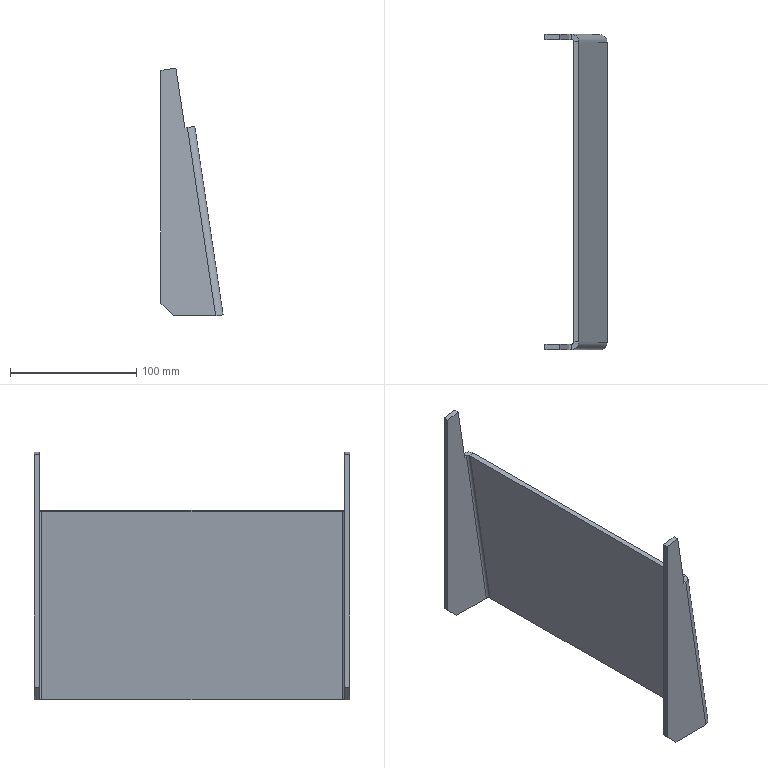Component | SolidWorks | THK-B1014SideStiffenerPlate-3 | 1 solid | 26 faces | box 49.3 x 250 x 196.5 mm | volume 195094 mm3 | plane 22 | cylinder 4 | commonest cylinder face diameters 12 x2 4 x2 | material Q235A
STEP:
#1=COLOUR_RGB('',0.7922,0.8196,0.9333);
#2=FILL_AREA_STYLE_COLOUR('',#1);
#3=FILL_AREA_STYLE('',(#2));
#4=SURFACE_STYLE_FILL_AREA(#3);
#5=SURFACE_SIDE_STYLE('',(#4));
#6=SURFACE_STYLE_USAGE(.BOTH.,#5);
#7=PRESENTATION_STYLE_ASSIGNMENT((#6));
#8=CARTESIAN_POINT('',(5.236,4.764,2.194));
#9=VERTEX_POINT('',#8);
#10=CARTESIAN_POINT('',(5.236,4.764,-5.079));
#11=VERTEX_POINT('',#10);
#12=CARTESIAN_POINT('',(5.236,4.764,-5.476));
#13=DIRECTION('',(0.,0.,-1.));
#14=VECTOR('',#13,39.37);
#15=LINE('',#12,#14);
#16=EDGE_CURVE('',#9,#11,#15,.T.);
#17=ORIENTED_EDGE('',*,*,#16,.T.);
#18=CARTESIAN_POINT('',(5.63,4.764,-5.472));
#19=VERTEX_POINT('',#18);
#20=CARTESIAN_POINT('',(5.63,4.764,-5.472));
#21=DIRECTION('',(0.7071,0.,-0.7071));
#22=VECTOR('',#21,39.37);
#23=LINE('',#20,#22);
#24=EDGE_CURVE('',#11,#19,#23,.T.);
#25=ORIENTED_EDGE('',*,*,#24,.T.);
#26=CARTESIAN_POINT('',(6.943,4.764,-5.472));
#27=VERTEX_POINT('',#26);
#28=CARTESIAN_POINT('',(7.183,4.764,-5.472));
#29=DIRECTION('',(1.,0.,0.));
#30=VECTOR('',#29,39.37);
#31=LINE('',#28,#30);
#32=EDGE_CURVE('',#19,#27,#31,.T.);
#33=ORIENTED_EDGE('',*,*,#32,.T.);
#34=CARTESIAN_POINT('',(6.062,4.764,0.4067));
#35=VERTEX_POINT('',#34);
#36=CARTESIAN_POINT('',(6.949,4.764,-5.511));
#37=DIRECTION('',(-0.1483,-0.,0.9889));
#38=VECTOR('',#37,39.37);
#39=LINE('',#36,#38);
#40=EDGE_CURVE('',#27,#35,#39,.T.);
#41=ORIENTED_EDGE('',*,*,#40,.T.);
#42=CARTESIAN_POINT('',(5.984,4.764,0.395));
#43=VERTEX_POINT('',#42);
#44=CARTESIAN_POINT('',(6.295,4.764,0.4417));
#45=DIRECTION('',(-0.9889,-0.,-0.1483));
#46=VECTOR('',#45,39.37);
#47=LINE('',#44,#46);
#48=EDGE_CURVE('',#35,#43,#47,.T.);
#49=ORIENTED_EDGE('',*,*,#48,.T.);
#50=CARTESIAN_POINT('',(5.703,4.764,2.264));
#51=VERTEX_POINT('',#50);
#52=CARTESIAN_POINT('',(6.871,4.764,-5.523));
#53=DIRECTION('',(-0.1483,-0.,0.9889));
#54=VECTOR('',#53,39.37);
#55=LINE('',#52,#54);
#56=EDGE_CURVE('',#43,#51,#55,.T.);
#57=ORIENTED_EDGE('',*,*,#56,.T.);
#58=CARTESIAN_POINT('',(6.015,4.764,2.311));
#59=DIRECTION('',(-0.9889,-0.,-0.1483));
#60=VECTOR('',#59,39.37);
#61=LINE('',#58,#60);
#62=EDGE_CURVE('',#51,#9,#61,.T.);
#63=ORIENTED_EDGE('',*,*,#62,.T.);
#64=EDGE_LOOP('',(#17,#25,#33,#41,#49,#57,#63));
#65=FACE_OUTER_BOUND('',#64,.T.);
#66=CARTESIAN_POINT('',(7.183,4.764,-5.476));
#67=DIRECTION('',(-0.,1.,0.));
#68=DIRECTION('',(0.9889,0.,0.1483));
#69=AXIS2_PLACEMENT_3D('',#66,#67,#68);
#70=PLANE('',#69);
#71=ADVANCED_FACE('',(#65),#70,.F.);
#72=CARTESIAN_POINT('',(6.943,4.921,-5.472));
#73=VERTEX_POINT('',#72);
#74=CARTESIAN_POINT('',(5.63,4.921,-5.472));
#75=VERTEX_POINT('',#74);
#76=CARTESIAN_POINT('',(6.943,4.921,-5.472));
#77=DIRECTION('',(-1.,-0.,-0.));
#78=VECTOR('',#77,39.37);
#79=LINE('',#76,#78);
#80=EDGE_CURVE('',#73,#75,#79,.T.);
#81=ORIENTED_EDGE('',*,*,#80,.T.);
#82=CARTESIAN_POINT('',(5.236,4.921,-5.079));
#83=VERTEX_POINT('',#82);
#84=CARTESIAN_POINT('',(6.408,4.921,-6.251));
#85=DIRECTION('',(-0.7071,-0.,0.7071));
#86=VECTOR('',#85,39.37);
#87=LINE('',#84,#86);
#88=EDGE_CURVE('',#75,#83,#87,.T.);
#89=ORIENTED_EDGE('',*,*,#88,.T.);
#90=CARTESIAN_POINT('',(5.236,4.921,2.194));
#91=VERTEX_POINT('',#90);
#92=CARTESIAN_POINT('',(5.236,4.921,-5.476));
#93=DIRECTION('',(0.,0.,-1.));
#94=VECTOR('',#93,39.37);
#95=LINE('',#92,#94);
#96=EDGE_CURVE('',#91,#83,#95,.T.);
#97=ORIENTED_EDGE('',*,*,#96,.F.);
#98=CARTESIAN_POINT('',(5.703,4.921,2.264));
#99=VERTEX_POINT('',#98);
#100=CARTESIAN_POINT('',(6.015,4.921,2.311));
#101=DIRECTION('',(-0.9889,-0.,-0.1483));
#102=VECTOR('',#101,39.37);
#103=LINE('',#100,#102);
#104=EDGE_CURVE('',#99,#91,#103,.T.);
#105=ORIENTED_EDGE('',*,*,#104,.F.);
#106=CARTESIAN_POINT('',(5.984,4.921,0.395));
#107=VERTEX_POINT('',#106);
#108=CARTESIAN_POINT('',(6.871,4.921,-5.523));
#109=DIRECTION('',(-0.1483,-0.,0.9889));
#110=VECTOR('',#109,39.37);
#111=LINE('',#108,#110);
#112=EDGE_CURVE('',#107,#99,#111,.T.);
#113=ORIENTED_EDGE('',*,*,#112,.F.);
#114=CARTESIAN_POINT('',(6.062,4.921,0.4067));
#115=VERTEX_POINT('',#114);
#116=CARTESIAN_POINT('',(6.295,4.921,0.4417));
#117=DIRECTION('',(-0.9889,-0.,-0.1483));
#118=VECTOR('',#117,39.37);
#119=LINE('',#116,#118);
#120=EDGE_CURVE('',#115,#107,#119,.T.);
#121=ORIENTED_EDGE('',*,*,#120,.F.);
#122=CARTESIAN_POINT('',(6.949,4.921,-5.511));
#123=DIRECTION('',(-0.1483,-0.,0.9889));
#124=VECTOR('',#123,39.37);
#125=LINE('',#122,#124);
#126=EDGE_CURVE('',#73,#115,#125,.T.);
#127=ORIENTED_EDGE('',*,*,#126,.F.);
#128=EDGE_LOOP('',(#81,#89,#97,#105,#113,#121,#127));
#129=FACE_OUTER_BOUND('',#128,.T.);
#130=CARTESIAN_POINT('',(7.183,4.921,-5.476));
#131=DIRECTION('',(-0.,1.,0.));
#132=DIRECTION('',(0.9889,0.,0.1483));
#133=AXIS2_PLACEMENT_3D('',#130,#131,#132);
#134=PLANE('',#133);
#135=ADVANCED_FACE('',(#129),#134,.T.);
#136=CARTESIAN_POINT('',(5.703,4.764,2.264));
#137=DIRECTION('',(-0.,1.,0.));
#138=VECTOR('',#137,39.37);
#139=LINE('',#136,#138);
#140=EDGE_CURVE('',#51,#99,#139,.T.);
#141=ORIENTED_EDGE('',*,*,#140,.T.);
#142=ORIENTED_EDGE('',*,*,#104,.T.);
#143=CARTESIAN_POINT('',(5.236,4.764,2.194));
#144=DIRECTION('',(-0.,1.,0.));
#145=VECTOR('',#144,39.37);
#146=LINE('',#143,#145);
#147=EDGE_CURVE('',#9,#91,#146,.T.);
#148=ORIENTED_EDGE('',*,*,#147,.F.);
#149=ORIENTED_EDGE('',*,*,#62,.F.);
#150=EDGE_LOOP('',(#141,#142,#148,#149));
#151=FACE_OUTER_BOUND('',#150,.T.);
#152=CARTESIAN_POINT('',(5.781,4.685,2.276));
#153=DIRECTION('',(0.1483,0.,-0.9889));
#154=DIRECTION('',(0.9889,0.,0.1483));
#155=AXIS2_PLACEMENT_3D('',#152,#153,#154);
#156=PLANE('',#155);
#157=ADVANCED_FACE('',(#151),#156,.F.);
#158=CARTESIAN_POINT('',(5.236,-4.921,2.194));
#159=VERTEX_POINT('',#158);
#160=CARTESIAN_POINT('',(5.703,-4.921,2.264));
#161=VERTEX_POINT('',#160);
#162=CARTESIAN_POINT('',(4.068,-4.921,2.019));
#163=DIRECTION('',(0.9889,0.,0.1483));
#164=VECTOR('',#163,39.37);
#165=LINE('',#162,#164);
#166=EDGE_CURVE('',#159,#161,#165,.T.);
#167=ORIENTED_EDGE('',*,*,#166,.T.);
#168=CARTESIAN_POINT('',(5.703,-4.764,2.264));
#169=VERTEX_POINT('',#168);
#170=CARTESIAN_POINT('',(5.703,-4.921,2.264));
#171=DIRECTION('',(-0.,1.,-0.));
#172=VECTOR('',#171,39.37);
#173=LINE('',#170,#172);
#174=EDGE_CURVE('',#161,#169,#173,.T.);
#175=ORIENTED_EDGE('',*,*,#174,.T.);
#176=CARTESIAN_POINT('',(5.236,-4.764,2.194));
#177=VERTEX_POINT('',#176);
#178=CARTESIAN_POINT('',(4.068,-4.764,2.019));
#179=DIRECTION('',(0.9889,0.,0.1483));
#180=VECTOR('',#179,39.37);
#181=LINE('',#178,#180);
#182=EDGE_CURVE('',#177,#169,#181,.T.);
#183=ORIENTED_EDGE('',*,*,#182,.F.);
#184=CARTESIAN_POINT('',(5.236,-4.764,2.194));
#185=DIRECTION('',(0.,-1.,0.));
#186=VECTOR('',#185,39.37);
#187=LINE('',#184,#186);
#188=EDGE_CURVE('',#177,#159,#187,.T.);
#189=ORIENTED_EDGE('',*,*,#188,.T.);
#190=EDGE_LOOP('',(#167,#175,#183,#189));
#191=FACE_OUTER_BOUND('',#190,.T.);
#192=CARTESIAN_POINT('',(5.859,-4.685,2.287));
#193=DIRECTION('',(-0.1483,-0.,0.9889));
#194=DIRECTION('',(-0.9889,-0.,-0.1483));
#195=AXIS2_PLACEMENT_3D('',#192,#193,#194);
#196=PLANE('',#195);
#197=ADVANCED_FACE('',(#191),#196,.T.);
#198=CARTESIAN_POINT('',(5.236,-4.921,-5.079));
#199=VERTEX_POINT('',#198);
#200=CARTESIAN_POINT('',(5.236,-4.921,-5.768));
#201=DIRECTION('',(-0.,0.,1.));
#202=VECTOR('',#201,39.37);
#203=LINE('',#200,#202);
#204=EDGE_CURVE('',#199,#159,#203,.T.);
#205=ORIENTED_EDGE('',*,*,#204,.F.);
#206=CARTESIAN_POINT('',(5.63,-4.921,-5.472));
#207=VERTEX_POINT('',#206);
#208=CARTESIAN_POINT('',(5.581,-4.921,-5.424));
#209=DIRECTION('',(0.7071,0.,-0.7071));
#210=VECTOR('',#209,39.37);
#211=LINE('',#208,#210);
#212=EDGE_CURVE('',#199,#207,#211,.T.);
#213=ORIENTED_EDGE('',*,*,#212,.T.);
#214=CARTESIAN_POINT('',(6.943,-4.921,-5.472));
#215=VERTEX_POINT('',#214);
#216=CARTESIAN_POINT('',(6.943,-4.921,-5.472));
#217=DIRECTION('',(-1.,-0.,-0.));
#218=VECTOR('',#217,39.37);
#219=LINE('',#216,#218);
#220=EDGE_CURVE('',#215,#207,#219,.T.);
#221=ORIENTED_EDGE('',*,*,#220,.F.);
#222=CARTESIAN_POINT('',(6.062,-4.921,0.4067));
#223=VERTEX_POINT('',#222);
#224=CARTESIAN_POINT('',(6.949,-4.921,-5.511));
#225=DIRECTION('',(-0.1483,-0.,0.9889));
#226=VECTOR('',#225,39.37);
#227=LINE('',#224,#226);
#228=EDGE_CURVE('',#215,#223,#227,.T.);
#229=ORIENTED_EDGE('',*,*,#228,.T.);
#230=CARTESIAN_POINT('',(5.984,-4.921,0.395));
#231=VERTEX_POINT('',#230);
#232=CARTESIAN_POINT('',(5.984,-4.921,0.395));
#233=DIRECTION('',(0.9889,0.,0.1483));
#234=VECTOR('',#233,39.37);
#235=LINE('',#232,#234);
#236=EDGE_CURVE('',#231,#223,#235,.T.);
#237=ORIENTED_EDGE('',*,*,#236,.F.);
#238=CARTESIAN_POINT('',(5.703,-4.921,2.264));
#239=DIRECTION('',(0.1483,0.,-0.9889));
#240=VECTOR('',#239,39.37);
#241=LINE('',#238,#240);
#242=EDGE_CURVE('',#161,#231,#241,.T.);
#243=ORIENTED_EDGE('',*,*,#242,.F.);
#244=ORIENTED_EDGE('',*,*,#166,.F.);
#245=EDGE_LOOP('',(#205,#213,#221,#229,#237,#243,#244));
#246=FACE_OUTER_BOUND('',#245,.T.);
#247=CARTESIAN_POINT('',(5.236,-4.921,-5.768));
#248=DIRECTION('',(0.,-1.,0.));
#249=DIRECTION('',(0.1483,0.,-0.9889));
#250=AXIS2_PLACEMENT_3D('',#247,#248,#249);
#251=PLANE('',#250);
#252=ADVANCED_FACE('',(#246),#251,.T.);
#253=CARTESIAN_POINT('',(6.943,-4.764,-5.472));
#254=VERTEX_POINT('',#253);
#255=CARTESIAN_POINT('',(5.63,-4.764,-5.472));
#256=VERTEX_POINT('',#255);
#257=CARTESIAN_POINT('',(5.236,-4.764,-5.472));
#258=DIRECTION('',(-1.,-0.,-0.));
#259=VECTOR('',#258,39.37);
#260=LINE('',#257,#259);
#261=EDGE_CURVE('',#254,#256,#260,.T.);
#262=ORIENTED_EDGE('',*,*,#261,.T.);
#263=CARTESIAN_POINT('',(5.236,-4.764,-5.079));
#264=VERTEX_POINT('',#263);
#265=CARTESIAN_POINT('',(5.63,-4.764,-5.472));
#266=DIRECTION('',(-0.7071,-0.,0.7071));
#267=VECTOR('',#266,39.37);
#268=LINE('',#265,#267);
#269=EDGE_CURVE('',#256,#264,#268,.T.);
#270=ORIENTED_EDGE('',*,*,#269,.T.);
#271=CARTESIAN_POINT('',(5.236,-4.764,-5.768));
#272=DIRECTION('',(-0.,0.,1.));
#273=VECTOR('',#272,39.37);
#274=LINE('',#271,#273);
#275=EDGE_CURVE('',#264,#177,#274,.T.);
#276=ORIENTED_EDGE('',*,*,#275,.T.);
#277=ORIENTED_EDGE('',*,*,#182,.T.);
#278=CARTESIAN_POINT('',(5.984,-4.764,0.395));
#279=VERTEX_POINT('',#278);
#280=CARTESIAN_POINT('',(6.871,-4.764,-5.523));
#281=DIRECTION('',(0.1483,0.,-0.9889));
#282=VECTOR('',#281,39.37);
#283=LINE('',#280,#282);
#284=EDGE_CURVE('',#169,#279,#283,.T.);
#285=ORIENTED_EDGE('',*,*,#284,.T.);
#286=CARTESIAN_POINT('',(6.062,-4.764,0.4067));
#287=VERTEX_POINT('',#286);
#288=CARTESIAN_POINT('',(4.349,-4.764,0.1497));
#289=DIRECTION('',(0.9889,0.,0.1483));
#290=VECTOR('',#289,39.37);
#291=LINE('',#288,#290);
#292=EDGE_CURVE('',#279,#287,#291,.T.);
#293=ORIENTED_EDGE('',*,*,#292,.T.);
#294=CARTESIAN_POINT('',(6.949,-4.764,-5.511));
#295=DIRECTION('',(-0.1483,-0.,0.9889));
#296=VECTOR('',#295,39.37);
#297=LINE('',#294,#296);
#298=EDGE_CURVE('',#254,#287,#297,.T.);
#299=ORIENTED_EDGE('',*,*,#298,.F.);
#300=EDGE_LOOP('',(#262,#270,#276,#277,#285,#293,#299));
#301=FACE_OUTER_BOUND('',#300,.T.);
#302=CARTESIAN_POINT('',(5.236,-4.764,-5.768));
#303=DIRECTION('',(0.,-1.,0.));
#304=DIRECTION('',(0.1483,0.,-0.9889));
#305=AXIS2_PLACEMENT_3D('',#302,#303,#304);
#306=PLANE('',#305);
#307=ADVANCED_FACE('',(#301),#306,.F.);
#308=CARTESIAN_POINT('',(7.177,4.685,-5.437));
#309=VERTEX_POINT('',#308);
#310=CARTESIAN_POINT('',(6.943,4.685,-5.472));
#311=DIRECTION('',(0.1483,0.,-0.9889));
#312=DIRECTION('',(-0.9889,-0.,-0.1483));
#313=AXIS2_PLACEMENT_3D('',#310,#311,#312);
#314=CIRCLE('',#313,0.2362);
#315=EDGE_CURVE('',#73,#309,#314,.T.);
#316=ORIENTED_EDGE('',*,*,#315,.F.);
#317=ORIENTED_EDGE('',*,*,#126,.T.);
#318=CARTESIAN_POINT('',(6.295,4.685,0.4417));
#319=VERTEX_POINT('',#318);
#320=CARTESIAN_POINT('',(6.062,4.685,0.4067));
#321=DIRECTION('',(-0.1483,-0.,0.9889));
#322=DIRECTION('',(0.9889,0.,0.1483));
#323=AXIS2_PLACEMENT_3D('',#320,#321,#322);
#324=CIRCLE('',#323,0.2362);
#325=EDGE_CURVE('',#319,#115,#324,.T.);
#326=ORIENTED_EDGE('',*,*,#325,.F.);
#327=CARTESIAN_POINT('',(7.183,4.685,-5.476));
#328=DIRECTION('',(-0.1483,-0.,0.9889));
#329=VECTOR('',#328,39.37);
#330=LINE('',#327,#329);
#331=EDGE_CURVE('',#309,#319,#330,.T.);
#332=ORIENTED_EDGE('',*,*,#331,.F.);
#333=EDGE_LOOP('',(#316,#317,#326,#332));
#334=FACE_OUTER_BOUND('',#333,.T.);
#335=CARTESIAN_POINT('',(6.949,4.685,-5.511));
#336=DIRECTION('',(-0.1483,-0.,0.9889));
#337=DIRECTION('',(-0.9889,-0.,-0.1483));
#338=AXIS2_PLACEMENT_3D('',#335,#336,#337);
#339=CYLINDRICAL_SURFACE('',#338,0.2362);
#340=ADVANCED_FACE('',(#334),#339,.T.);
#341=CARTESIAN_POINT('',(7.177,-4.685,-5.437));
#342=VERTEX_POINT('',#341);
#343=CARTESIAN_POINT('',(7.177,4.921,-5.437));
#344=DIRECTION('',(0.,-1.,0.));
#345=VECTOR('',#344,39.37);
#346=LINE('',#343,#345);
#347=EDGE_CURVE('',#309,#342,#346,.T.);
#348=ORIENTED_EDGE('',*,*,#347,.F.);
#349=ORIENTED_EDGE('',*,*,#331,.T.);
#350=CARTESIAN_POINT('',(6.295,-4.685,0.4417));
#351=VERTEX_POINT('',#350);
#352=CARTESIAN_POINT('',(6.295,4.921,0.4417));
#353=DIRECTION('',(0.,-1.,0.));
#354=VECTOR('',#353,39.37);
#355=LINE('',#352,#354);
#356=EDGE_CURVE('',#319,#351,#355,.T.);
#357=ORIENTED_EDGE('',*,*,#356,.T.);
#358=CARTESIAN_POINT('',(7.183,-4.685,-5.476));
#359=DIRECTION('',(-0.1483,-0.,0.9889));
#360=VECTOR('',#359,39.37);
#361=LINE('',#358,#360);
#362=EDGE_CURVE('',#342,#351,#361,.T.);
#363=ORIENTED_EDGE('',*,*,#362,.F.);
#364=EDGE_LOOP('',(#348,#349,#357,#363));
#365=FACE_OUTER_BOUND('',#364,.T.);
#366=CARTESIAN_POINT('',(7.183,-4.921,-5.476));
#367=DIRECTION('',(0.9889,0.,0.1483));
#368=DIRECTION('',(0.,-1.,-0.));
#369=AXIS2_PLACEMENT_3D('',#366,#367,#368);
#370=PLANE('',#369);
#371=ADVANCED_FACE('',(#365),#370,.T.);
#372=CARTESIAN_POINT('',(6.943,-4.685,-5.472));
#373=DIRECTION('',(0.1483,0.,-0.9889));
#374=DIRECTION('',(-0.9889,-0.,-0.1483));
#375=AXIS2_PLACEMENT_3D('',#372,#373,#374);
#376=CIRCLE('',#375,0.2362);
#377=EDGE_CURVE('',#342,#215,#376,.T.);
#378=ORIENTED_EDGE('',*,*,#377,.F.);
#379=ORIENTED_EDGE('',*,*,#362,.T.);
#380=CARTESIAN_POINT('',(6.062,-4.685,0.4067));
#381=DIRECTION('',(-0.1483,-0.,0.9889));
#382=DIRECTION('',(0.9889,0.,0.1483));
#383=AXIS2_PLACEMENT_3D('',#380,#381,#382);
#384=CIRCLE('',#383,0.2362);
#385=EDGE_CURVE('',#223,#351,#384,.T.);
#386=ORIENTED_EDGE('',*,*,#385,.F.);
#387=ORIENTED_EDGE('',*,*,#228,.F.);
#388=EDGE_LOOP('',(#378,#379,#386,#387));
#389=FACE_OUTER_BOUND('',#388,.T.);
#390=CARTESIAN_POINT('',(6.949,-4.685,-5.511));
#391=DIRECTION('',(-0.1483,-0.,0.9889));
#392=DIRECTION('',(-0.9889,-0.,-0.1483));
#393=AXIS2_PLACEMENT_3D('',#390,#391,#392);
#394=CYLINDRICAL_SURFACE('',#393,0.2362);
#395=ADVANCED_FACE('',(#389),#394,.T.);
#396=CARTESIAN_POINT('',(7.021,-4.685,-5.461));
#397=VERTEX_POINT('',#396);
#398=CARTESIAN_POINT('',(6.14,-4.685,0.4183));
#399=VERTEX_POINT('',#398);
#400=CARTESIAN_POINT('',(7.027,-4.685,-5.5));
#401=DIRECTION('',(-0.1483,-0.,0.9889));
#402=VECTOR('',#401,39.37);
#403=LINE('',#400,#402);
#404=EDGE_CURVE('',#397,#399,#403,.T.);
#405=ORIENTED_EDGE('',*,*,#404,.F.);
#406=CARTESIAN_POINT('',(6.943,-4.685,-5.472));
#407=DIRECTION('',(0.1483,0.,-0.9889));
#408=DIRECTION('',(-0.9889,0.,-0.1483));
#409=AXIS2_PLACEMENT_3D('',#406,#407,#408);
#410=CIRCLE('',#409,0.07874);
#411=EDGE_CURVE('',#397,#254,#410,.T.);
#412=ORIENTED_EDGE('',*,*,#411,.T.);
#413=ORIENTED_EDGE('',*,*,#298,.T.);
#414=CARTESIAN_POINT('',(6.062,-4.685,0.4067));
#415=DIRECTION('',(-0.1483,-0.,0.9889));
#416=DIRECTION('',(-0.9889,0.,-0.1483));
#417=AXIS2_PLACEMENT_3D('',#414,#415,#416);
#418=CIRCLE('',#417,0.07874);
#419=EDGE_CURVE('',#287,#399,#418,.T.);
#420=ORIENTED_EDGE('',*,*,#419,.T.);
#421=EDGE_LOOP('',(#405,#412,#413,#420));
#422=FACE_OUTER_BOUND('',#421,.T.);
#423=CARTESIAN_POINT('',(6.949,-4.685,-5.511));
#424=DIRECTION('',(-0.1483,-0.,0.9889));
#425=DIRECTION('',(-0.9889,0.,-0.1483));
#426=AXIS2_PLACEMENT_3D('',#423,#424,#425);
#427=CYLINDRICAL_SURFACE('',#426,0.07874);
#428=ADVANCED_FACE('',(#422),#427,.F.);
#429=CARTESIAN_POINT('',(7.021,4.685,-5.461));
#430=VERTEX_POINT('',#429);
#431=CARTESIAN_POINT('',(6.14,4.685,0.4183));
#432=VERTEX_POINT('',#431);
#433=CARTESIAN_POINT('',(7.027,4.685,-5.5));
#434=DIRECTION('',(-0.1483,-0.,0.9889));
#435=VECTOR('',#434,39.37);
#436=LINE('',#433,#435);
#437=EDGE_CURVE('',#430,#432,#436,.T.);
#438=ORIENTED_EDGE('',*,*,#437,.F.);
#439=CARTESIAN_POINT('',(7.021,-4.921,-5.461));
#440=DIRECTION('',(0.,-1.,-0.));
#441=VECTOR('',#440,39.37);
#442=LINE('',#439,#441);
#443=EDGE_CURVE('',#430,#397,#442,.T.);
#444=ORIENTED_EDGE('',*,*,#443,.T.);
#445=ORIENTED_EDGE('',*,*,#404,.T.);
#446=CARTESIAN_POINT('',(6.14,-4.921,0.4183));
#447=DIRECTION('',(0.,-1.,-0.));
#448=VECTOR('',#447,39.37);
#449=LINE('',#446,#448);
#450=EDGE_CURVE('',#432,#399,#449,.T.);
#451=ORIENTED_EDGE('',*,*,#450,.F.);
#452=EDGE_LOOP('',(#438,#444,#445,#451));
#453=FACE_OUTER_BOUND('',#452,.T.);
#454=CARTESIAN_POINT('',(7.027,-4.921,-5.5));
#455=DIRECTION('',(0.9889,0.,0.1483));
#456=DIRECTION('',(0.,-1.,-0.));
#457=AXIS2_PLACEMENT_3D('',#454,#455,#456);
#458=PLANE('',#457);
#459=ADVANCED_FACE('',(#453),#458,.F.);
#460=ORIENTED_EDGE('',*,*,#40,.F.);
#461=CARTESIAN_POINT('',(6.943,4.685,-5.472));
#462=DIRECTION('',(0.1483,0.,-0.9889));
#463=DIRECTION('',(-0.9889,0.,-0.1483));
#464=AXIS2_PLACEMENT_3D('',#461,#462,#463);
#465=CIRCLE('',#464,0.07874);
#466=EDGE_CURVE('',#27,#430,#465,.T.);
#467=ORIENTED_EDGE('',*,*,#466,.T.);
#468=ORIENTED_EDGE('',*,*,#437,.T.);
#469=CARTESIAN_POINT('',(6.062,4.685,0.4067));
#470=DIRECTION('',(-0.1483,-0.,0.9889));
#471=DIRECTION('',(-0.9889,0.,-0.1483));
#472=AXIS2_PLACEMENT_3D('',#469,#470,#471);
#473=CIRCLE('',#472,0.07874);
#474=EDGE_CURVE('',#432,#35,#473,.T.);
#475=ORIENTED_EDGE('',*,*,#474,.T.);
#476=EDGE_LOOP('',(#460,#467,#468,#475));
#477=FACE_OUTER_BOUND('',#476,.T.);
#478=CARTESIAN_POINT('',(6.949,4.685,-5.511));
#479=DIRECTION('',(-0.1483,-0.,0.9889));
#480=DIRECTION('',(-0.9889,0.,-0.1483));
#481=AXIS2_PLACEMENT_3D('',#478,#479,#480);
#482=CYLINDRICAL_SURFACE('',#481,0.07874);
#483=ADVANCED_FACE('',(#477),#482,.F.);
#484=ORIENTED_EDGE('',*,*,#275,.F.);
#485=CARTESIAN_POINT('',(5.236,-4.921,-5.079));
#486=DIRECTION('',(0.,-1.,0.));
#487=VECTOR('',#486,39.37);
#488=LINE('',#485,#487);
#489=EDGE_CURVE('',#264,#199,#488,.T.);
#490=ORIENTED_EDGE('',*,*,#489,.T.);
#491=ORIENTED_EDGE('',*,*,#204,.T.);
#492=ORIENTED_EDGE('',*,*,#188,.F.);
#493=EDGE_LOOP('',(#484,#490,#491,#492));
#494=FACE_OUTER_BOUND('',#493,.T.);
#495=CARTESIAN_POINT('',(5.236,-4.764,-5.768));
#496=DIRECTION('',(1.,0.,0.));
#497=DIRECTION('',(-0.,0.,1.));
#498=AXIS2_PLACEMENT_3D('',#495,#496,#497);
#499=PLANE('',#498);
#500=ADVANCED_FACE('',(#494),#499,.F.);
#501=ORIENTED_EDGE('',*,*,#96,.T.);
#502=CARTESIAN_POINT('',(5.236,4.764,-5.079));
#503=DIRECTION('',(0.,-1.,0.));
#504=VECTOR('',#503,39.37);
#505=LINE('',#502,#504);
#506=EDGE_CURVE('',#83,#11,#505,.T.);
#507=ORIENTED_EDGE('',*,*,#506,.T.);
#508=ORIENTED_EDGE('',*,*,#16,.F.);
#509=ORIENTED_EDGE('',*,*,#147,.T.);
#510=EDGE_LOOP('',(#501,#507,#508,#509));
#511=FACE_OUTER_BOUND('',#510,.T.);
#512=CARTESIAN_POINT('',(5.236,4.764,-5.476));
#513=DIRECTION('',(1.,0.,0.));
#514=DIRECTION('',(0.,0.,-1.));
#515=AXIS2_PLACEMENT_3D('',#512,#513,#514);
#516=PLANE('',#515);
#517=ADVANCED_FACE('',(#511),#516,.F.);
#518=ORIENTED_EDGE('',*,*,#140,.F.);
#519=ORIENTED_EDGE('',*,*,#56,.F.);
#520=CARTESIAN_POINT('',(5.984,4.764,0.395));
#521=DIRECTION('',(-0.,1.,0.));
#522=VECTOR('',#521,39.37);
#523=LINE('',#520,#522);
#524=EDGE_CURVE('',#43,#107,#523,.T.);
#525=ORIENTED_EDGE('',*,*,#524,.T.);
#526=ORIENTED_EDGE('',*,*,#112,.T.);
#527=EDGE_LOOP('',(#518,#519,#525,#526));
#528=FACE_OUTER_BOUND('',#527,.T.);
#529=CARTESIAN_POINT('',(6.871,4.764,-5.523));
#530=DIRECTION('',(-0.9889,-0.,-0.1483));
#531=DIRECTION('',(-0.1483,-0.,0.9889));
#532=AXIS2_PLACEMENT_3D('',#529,#530,#531);
#533=PLANE('',#532);
#534=ADVANCED_FACE('',(#528),#533,.F.);
#535=ORIENTED_EDGE('',*,*,#524,.F.);
#536=ORIENTED_EDGE('',*,*,#48,.F.);
#537=CARTESIAN_POINT('',(6.062,4.764,0.4067));
#538=DIRECTION('',(-0.,1.,0.));
#539=VECTOR('',#538,39.37);
#540=LINE('',#537,#539);
#541=EDGE_CURVE('',#35,#115,#540,.T.);
#542=ORIENTED_EDGE('',*,*,#541,.T.);
#543=ORIENTED_EDGE('',*,*,#120,.T.);
#544=EDGE_LOOP('',(#535,#536,#542,#543));
#545=FACE_OUTER_BOUND('',#544,.T.);
#546=CARTESIAN_POINT('',(6.295,4.764,0.4417));
#547=DIRECTION('',(0.1483,0.,-0.9889));
#548=DIRECTION('',(-0.9889,-0.,-0.1483));
#549=AXIS2_PLACEMENT_3D('',#546,#547,#548);
#550=PLANE('',#549);
#551=ADVANCED_FACE('',(#545),#550,.F.);
#552=ORIENTED_EDGE('',*,*,#356,.F.);
#553=CARTESIAN_POINT('',(6.295,4.685,0.4417));
#554=DIRECTION('',(-0.9889,-0.,-0.1483));
#555=VECTOR('',#554,39.37);
#556=LINE('',#553,#555);
#557=EDGE_CURVE('',#319,#432,#556,.T.);
#558=ORIENTED_EDGE('',*,*,#557,.T.);
#559=ORIENTED_EDGE('',*,*,#450,.T.);
#560=CARTESIAN_POINT('',(6.295,-4.685,0.4417));
#561=DIRECTION('',(-0.9889,-0.,-0.1483));
#562=VECTOR('',#561,39.37);
#563=LINE('',#560,#562);
#564=EDGE_CURVE('',#351,#399,#563,.T.);
#565=ORIENTED_EDGE('',*,*,#564,.F.);
#566=EDGE_LOOP('',(#552,#558,#559,#565));
#567=FACE_OUTER_BOUND('',#566,.T.);
#568=CARTESIAN_POINT('',(6.295,4.921,0.4417));
#569=DIRECTION('',(-0.1483,-0.,0.9889));
#570=DIRECTION('',(0.,-1.,0.));
#571=AXIS2_PLACEMENT_3D('',#568,#569,#570);
#572=PLANE('',#571);
#573=ADVANCED_FACE('',(#567),#572,.T.);
#574=ORIENTED_EDGE('',*,*,#174,.F.);
#575=ORIENTED_EDGE('',*,*,#242,.T.);
#576=CARTESIAN_POINT('',(5.984,-4.921,0.395));
#577=DIRECTION('',(-0.,1.,-0.));
#578=VECTOR('',#577,39.37);
#579=LINE('',#576,#578);
#580=EDGE_CURVE('',#231,#279,#579,.T.);
#581=ORIENTED_EDGE('',*,*,#580,.T.);
#582=ORIENTED_EDGE('',*,*,#284,.F.);
#583=EDGE_LOOP('',(#574,#575,#581,#582));
#584=FACE_OUTER_BOUND('',#583,.T.);
#585=CARTESIAN_POINT('',(5.703,-4.921,2.264));
#586=DIRECTION('',(-0.9889,-0.,-0.1483));
#587=DIRECTION('',(0.1483,0.,-0.9889));
#588=AXIS2_PLACEMENT_3D('',#585,#586,#587);
#589=PLANE('',#588);
#590=ADVANCED_FACE('',(#584),#589,.F.);
#591=ORIENTED_EDGE('',*,*,#236,.T.);
#592=CARTESIAN_POINT('',(6.062,-4.921,0.4067));
#593=DIRECTION('',(-0.,1.,-0.));
#594=VECTOR('',#593,39.37);
#595=LINE('',#592,#594);
#596=EDGE_CURVE('',#223,#287,#595,.T.);
#597=ORIENTED_EDGE('',*,*,#596,.T.);
#598=ORIENTED_EDGE('',*,*,#292,.F.);
#599=ORIENTED_EDGE('',*,*,#580,.F.);
#600=EDGE_LOOP('',(#591,#597,#598,#599));
#601=FACE_OUTER_BOUND('',#600,.T.);
#602=CARTESIAN_POINT('',(5.984,-4.921,0.395));
#603=DIRECTION('',(0.1483,0.,-0.9889));
#604=DIRECTION('',(0.9889,0.,0.1483));
#605=AXIS2_PLACEMENT_3D('',#602,#603,#604);
#606=PLANE('',#605);
#607=ADVANCED_FACE('',(#601),#606,.F.);
#608=ORIENTED_EDGE('',*,*,#385,.T.);
#609=ORIENTED_EDGE('',*,*,#564,.T.);
#610=ORIENTED_EDGE('',*,*,#419,.F.);
#611=ORIENTED_EDGE('',*,*,#596,.F.);
#612=EDGE_LOOP('',(#608,#609,#610,#611));
#613=FACE_OUTER_BOUND('',#612,.T.);
#614=CARTESIAN_POINT('',(6.062,-4.685,0.4067));
#615=DIRECTION('',(-0.1483,-0.,0.9889));
#616=DIRECTION('',(-0.9889,-0.,-0.1483));
#617=AXIS2_PLACEMENT_3D('',#614,#615,#616);
#618=PLANE('',#617);
#619=ADVANCED_FACE('',(#613),#618,.T.);
#620=ORIENTED_EDGE('',*,*,#325,.T.);
#621=ORIENTED_EDGE('',*,*,#541,.F.);
#622=ORIENTED_EDGE('',*,*,#474,.F.);
#623=ORIENTED_EDGE('',*,*,#557,.F.);
#624=EDGE_LOOP('',(#620,#621,#622,#623));
#625=FACE_OUTER_BOUND('',#624,.T.);
#626=CARTESIAN_POINT('',(6.062,4.685,0.4067));
#627=DIRECTION('',(-0.1483,-0.,0.9889));
#628=DIRECTION('',(-0.9889,-0.,-0.1483));
#629=AXIS2_PLACEMENT_3D('',#626,#627,#628);
#630=PLANE('',#629);
#631=ADVANCED_FACE('',(#625),#630,.T.);
#632=ORIENTED_EDGE('',*,*,#315,.T.);
#633=ORIENTED_EDGE('',*,*,#347,.T.);
#634=ORIENTED_EDGE('',*,*,#377,.T.);
#635=CARTESIAN_POINT('',(6.943,4.921,-5.472));
#636=DIRECTION('',(0.,-1.,0.));
#637=VECTOR('',#636,39.37);
#638=LINE('',#635,#637);
#639=EDGE_CURVE('',#254,#215,#638,.T.);
#640=ORIENTED_EDGE('',*,*,#639,.F.);
#641=ORIENTED_EDGE('',*,*,#411,.F.);
#642=ORIENTED_EDGE('',*,*,#443,.F.);
#643=ORIENTED_EDGE('',*,*,#466,.F.);
#644=CARTESIAN_POINT('',(6.943,4.921,-5.472));
#645=DIRECTION('',(0.,-1.,0.));
#646=VECTOR('',#645,39.37);
#647=LINE('',#644,#646);
#648=EDGE_CURVE('',#73,#27,#647,.T.);
#649=ORIENTED_EDGE('',*,*,#648,.F.);
#650=EDGE_LOOP('',(#632,#633,#634,#640,#641,#642,#643,#649));
#651=FACE_OUTER_BOUND('',#650,.T.);
#652=CARTESIAN_POINT('',(6.943,4.921,-5.472));
#653=DIRECTION('',(-0.1483,-0.,0.9889));
#654=DIRECTION('',(-0.9889,-0.,-0.1483));
#655=AXIS2_PLACEMENT_3D('',#652,#653,#654);
#656=PLANE('',#655);
#657=ADVANCED_FACE('',(#651),#656,.F.);
#658=ORIENTED_EDGE('',*,*,#220,.T.);
#659=CARTESIAN_POINT('',(5.63,-4.764,-5.472));
#660=DIRECTION('',(-0.,1.,-0.));
#661=VECTOR('',#660,39.37);
#662=LINE('',#659,#661);
#663=EDGE_CURVE('',#207,#256,#662,.T.);
#664=ORIENTED_EDGE('',*,*,#663,.T.);
#665=ORIENTED_EDGE('',*,*,#261,.F.);
#666=ORIENTED_EDGE('',*,*,#639,.T.);
#667=EDGE_LOOP('',(#658,#664,#665,#666));
#668=FACE_OUTER_BOUND('',#667,.T.);
#669=CARTESIAN_POINT('',(6.943,4.921,-5.472));
#670=DIRECTION('',(-0.,0.,1.));
#671=DIRECTION('',(-1.,-0.,-0.));
#672=AXIS2_PLACEMENT_3D('',#669,#670,#671);
#673=PLANE('',#672);
#674=ADVANCED_FACE('',(#668),#673,.F.);
#675=ORIENTED_EDGE('',*,*,#32,.F.);
#676=CARTESIAN_POINT('',(5.63,4.921,-5.472));
#677=DIRECTION('',(-0.,1.,-0.));
#678=VECTOR('',#677,39.37);
#679=LINE('',#676,#678);
#680=EDGE_CURVE('',#19,#75,#679,.T.);
#681=ORIENTED_EDGE('',*,*,#680,.T.);
#682=ORIENTED_EDGE('',*,*,#80,.F.);
#683=ORIENTED_EDGE('',*,*,#648,.T.);
#684=EDGE_LOOP('',(#675,#681,#682,#683));
#685=FACE_OUTER_BOUND('',#684,.T.);
#686=CARTESIAN_POINT('',(6.943,4.921,-5.472));
#687=DIRECTION('',(-0.,0.,1.));
#688=DIRECTION('',(-1.,-0.,-0.));
#689=AXIS2_PLACEMENT_3D('',#686,#687,#688);
#690=PLANE('',#689);
#691=ADVANCED_FACE('',(#685),#690,.F.);
#692=ORIENTED_EDGE('',*,*,#24,.F.);
#693=ORIENTED_EDGE('',*,*,#506,.F.);
#694=ORIENTED_EDGE('',*,*,#88,.F.);
#695=ORIENTED_EDGE('',*,*,#680,.F.);
#696=EDGE_LOOP('',(#692,#693,#694,#695));
#697=FACE_OUTER_BOUND('',#696,.T.);
#698=CARTESIAN_POINT('',(5.63,4.921,-5.472));
#699=DIRECTION('',(0.7071,0.,0.7071));
#700=DIRECTION('',(-0.,1.,-0.));
#701=AXIS2_PLACEMENT_3D('',#698,#699,#700);
#702=PLANE('',#701);
#703=ADVANCED_FACE('',(#697),#702,.F.);
#704=ORIENTED_EDGE('',*,*,#212,.F.);
#705=ORIENTED_EDGE('',*,*,#489,.F.);
#706=ORIENTED_EDGE('',*,*,#269,.F.);
#707=ORIENTED_EDGE('',*,*,#663,.F.);
#708=EDGE_LOOP('',(#704,#705,#706,#707));
#709=FACE_OUTER_BOUND('',#708,.T.);
#710=CARTESIAN_POINT('',(5.63,4.921,-5.472));
#711=DIRECTION('',(0.7071,0.,0.7071));
#712=DIRECTION('',(-0.,1.,-0.));
#713=AXIS2_PLACEMENT_3D('',#710,#711,#712);
#714=PLANE('',#713);
#715=ADVANCED_FACE('',(#709),#714,.F.);
#716=CLOSED_SHELL('',(#71,#135,#157,#197,#252,#307,#340,#371,#395,#428,#459,#483,#500,#517,#534,#551,#573,#590,#607,#619,#631,#657,#674,#691,#703,#715));
#717=MANIFOLD_SOLID_BREP('',#716);
#718=STYLED_ITEM('',(#7),#717);
#719=(LENGTH_UNIT()NAMED_UNIT(*)SI_UNIT($,.METRE.));
#720=LENGTH_MEASURE_WITH_UNIT(LENGTH_MEASURE(0.0254),#719);
#721=DIMENSIONAL_EXPONENTS(1.,0.,0.,0.,0.,0.,0.);
#722=(CONVERSION_BASED_UNIT('',#720)LENGTH_UNIT()NAMED_UNIT(#721));
#723=UNCERTAINTY_MEASURE_WITH_UNIT(LENGTH_MEASURE(0.00001),#722,'','');
#724=(NAMED_UNIT(*)PLANE_ANGLE_UNIT()SI_UNIT($,.RADIAN.));
#725=(NAMED_UNIT(*)SI_UNIT($,.STERADIAN.)SOLID_ANGLE_UNIT());
#726=(GEOMETRIC_REPRESENTATION_CONTEXT(3)GLOBAL_UNCERTAINTY_ASSIGNED_CONTEXT((#723))GLOBAL_UNIT_ASSIGNED_CONTEXT((#722,#724,#725))REPRESENTATION_CONTEXT('',''));
#727=MECHANICAL_DESIGN_GEOMETRIC_PRESENTATION_REPRESENTATION('',(#718),#726);
#728=PRESENTATION_LAYER_ASSIGNMENT('','',(#718));
#729=CARTESIAN_POINT('',(0.,0.,0.));
#730=DIRECTION('',(0.,0.,1.));
#731=DIRECTION('',(1.,0.,0.));
#732=AXIS2_PLACEMENT_3D('',#729,#730,#731);
#733=(LENGTH_UNIT()NAMED_UNIT(*)SI_UNIT($,.METRE.));
#734=LENGTH_MEASURE_WITH_UNIT(LENGTH_MEASURE(0.0254),#733);
#735=DIMENSIONAL_EXPONENTS(1.,0.,0.,0.,0.,0.,0.);
#736=(CONVERSION_BASED_UNIT('',#734)LENGTH_UNIT()NAMED_UNIT(#735));
#737=UNCERTAINTY_MEASURE_WITH_UNIT(LENGTH_MEASURE(0.00001),#736,'','');
#738=(NAMED_UNIT(*)PLANE_ANGLE_UNIT()SI_UNIT($,.RADIAN.));
#739=(NAMED_UNIT(*)SI_UNIT($,.STERADIAN.)SOLID_ANGLE_UNIT());
#740=(GEOMETRIC_REPRESENTATION_CONTEXT(3)GLOBAL_UNCERTAINTY_ASSIGNED_CONTEXT((#737))GLOBAL_UNIT_ASSIGNED_CONTEXT((#736,#738,#739))REPRESENTATION_CONTEXT('',''));
#741=ADVANCED_BREP_SHAPE_REPRESENTATION('',(#717,#732),#740);